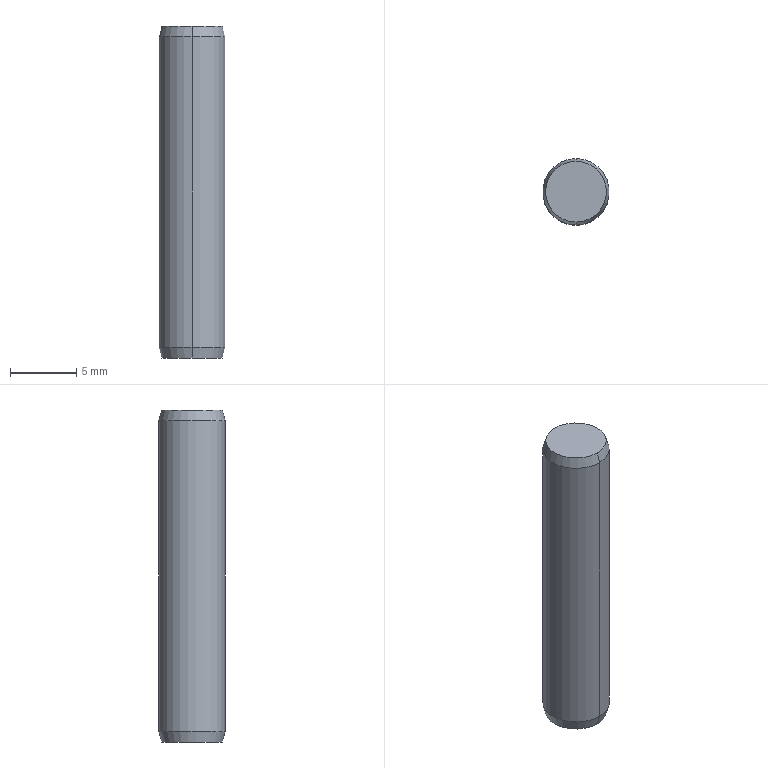Component | NX | PIN_M5X25 | 1 solid | 8 faces | box 5 x 5 x 25 mm | volume 488 mm3 | cone 4 | cylinder 2 | plane 2 | commonest cylinder face diameters 5 x2
STEP:
#1=CARTESIAN_POINT('',(0.,0.,0.));
#2=DIRECTION('',(0.,0.,1.));
#3=DIRECTION('',(1.,0.,0.));
#4=AXIS2_PLACEMENT_3D('',#1,#2,#3);
#5=CARTESIAN_POINT('',(-222.594,88.985,75.8));
#6=VERTEX_POINT('',#5);
#7=CARTESIAN_POINT('',(-222.594,88.77,75.));
#8=VERTEX_POINT('',#7);
#9=CARTESIAN_POINT('',(-222.594,88.878,75.4));
#10=DIRECTION('',(0.,-0.2588,-0.9659));
#11=VECTOR('',#10,1.);
#12=LINE('',#9,#11);
#13=CARTESIAN_POINT('',(-222.594,86.485,75.4));
#14=DIRECTION('',(0.,0.,1.));
#15=DIRECTION('',(0.,-1.,0.));
#16=AXIS2_PLACEMENT_3D('',#13,#14,#15);
#17=CONICAL_SURFACE('',#16,2.393,0.2618);
#18=CARTESIAN_POINT('',(3.142,-0.));
#19=DIRECTION('',(0.,-1.));
#20=VECTOR('',#19,1.);
#21=LINE('',#18,#20);
#22=(GEOMETRIC_REPRESENTATION_CONTEXT(2)PARAMETRIC_REPRESENTATION_CONTEXT()REPRESENTATION_CONTEXT('',''));
#23=DEFINITIONAL_REPRESENTATION('',(#21),#22);
#24=PCURVE('',#17,#23);
#25=CARTESIAN_POINT('',(-222.594,86.485,75.4));
#26=DIRECTION('',(0.,0.,1.));
#27=DIRECTION('',(0.,-1.,0.));
#28=AXIS2_PLACEMENT_3D('',#25,#26,#27);
#29=CONICAL_SURFACE('',#28,2.393,0.2618);
#30=CARTESIAN_POINT('',(3.142,-0.));
#31=DIRECTION('',(0.,-1.));
#32=VECTOR('',#31,1.);
#33=LINE('',#30,#32);
#34=(GEOMETRIC_REPRESENTATION_CONTEXT(2)PARAMETRIC_REPRESENTATION_CONTEXT()REPRESENTATION_CONTEXT('',''));
#35=DEFINITIONAL_REPRESENTATION('',(#33),#34);
#36=PCURVE('',#29,#35);
#37=SURFACE_CURVE('',#12,(#24,#36),.PCURVE_S1.);
#38=EDGE_CURVE('',#6,#8,#37,.T.);
#39=ORIENTED_EDGE('',*,*,#38,.F.);
#40=CARTESIAN_POINT('',(-222.594,83.985,75.8));
#41=VERTEX_POINT('',#40);
#42=CARTESIAN_POINT('',(-222.594,86.485,75.8));
#43=DIRECTION('',(0.,0.,-1.));
#44=DIRECTION('',(0.,1.,0.));
#45=AXIS2_PLACEMENT_3D('',#42,#43,#44);
#46=CIRCLE('',#45,2.5);
#47=CARTESIAN_POINT('',(3.142,0.4));
#48=DIRECTION('',(-1.,0.));
#49=VECTOR('',#48,1.);
#50=LINE('',#47,#49);
#51=(GEOMETRIC_REPRESENTATION_CONTEXT(2)PARAMETRIC_REPRESENTATION_CONTEXT()REPRESENTATION_CONTEXT('',''));
#52=DEFINITIONAL_REPRESENTATION('',(#50),#51);
#53=PCURVE('',#17,#52);
#54=CARTESIAN_POINT('',(-222.594,86.485,90.));
#55=DIRECTION('',(0.,0.,-1.));
#56=DIRECTION('',(0.,-1.,0.));
#57=AXIS2_PLACEMENT_3D('',#54,#55,#56);
#58=CYLINDRICAL_SURFACE('',#57,2.5);
#59=CARTESIAN_POINT('',(3.142,14.2));
#60=DIRECTION('',(1.,0.));
#61=VECTOR('',#60,1.);
#62=LINE('',#59,#61);
#63=(GEOMETRIC_REPRESENTATION_CONTEXT(2)PARAMETRIC_REPRESENTATION_CONTEXT()REPRESENTATION_CONTEXT('',''));
#64=DEFINITIONAL_REPRESENTATION('',(#62),#63);
#65=PCURVE('',#58,#64);
#66=SURFACE_CURVE('',#46,(#53,#65),.PCURVE_S1.);
#67=EDGE_CURVE('',#6,#41,#66,.T.);
#68=ORIENTED_EDGE('',*,*,#67,.T.);
#69=CARTESIAN_POINT('',(-222.594,84.199,75.));
#70=VERTEX_POINT('',#69);
#71=CARTESIAN_POINT('',(-222.594,84.092,75.4));
#72=DIRECTION('',(0.,-0.2588,0.9659));
#73=VECTOR('',#72,1.);
#74=LINE('',#71,#73);
#75=CARTESIAN_POINT('',(0.,0.));
#76=DIRECTION('',(0.,1.));
#77=VECTOR('',#76,1.);
#78=LINE('',#75,#77);
#79=(GEOMETRIC_REPRESENTATION_CONTEXT(2)PARAMETRIC_REPRESENTATION_CONTEXT()REPRESENTATION_CONTEXT('',''));
#80=DEFINITIONAL_REPRESENTATION('',(#78),#79);
#81=PCURVE('',#17,#80);
#82=CARTESIAN_POINT('',(6.283,0.));
#83=DIRECTION('',(0.,1.));
#84=VECTOR('',#83,1.);
#85=LINE('',#82,#84);
#86=(GEOMETRIC_REPRESENTATION_CONTEXT(2)PARAMETRIC_REPRESENTATION_CONTEXT()REPRESENTATION_CONTEXT('',''));
#87=DEFINITIONAL_REPRESENTATION('',(#85),#86);
#88=PCURVE('',#29,#87);
#89=SURFACE_CURVE('',#74,(#81,#88),.PCURVE_S1.);
#90=EDGE_CURVE('',#70,#41,#89,.T.);
#91=ORIENTED_EDGE('',*,*,#90,.F.);
#92=CARTESIAN_POINT('',(-222.594,86.485,75.));
#93=DIRECTION('',(0.,0.,-1.));
#94=DIRECTION('',(0.,1.,0.));
#95=AXIS2_PLACEMENT_3D('',#92,#93,#94);
#96=CIRCLE('',#95,2.286);
#97=CARTESIAN_POINT('',(3.142,-0.4));
#98=DIRECTION('',(-1.,0.));
#99=VECTOR('',#98,1.);
#100=LINE('',#97,#99);
#101=(GEOMETRIC_REPRESENTATION_CONTEXT(2)PARAMETRIC_REPRESENTATION_CONTEXT()REPRESENTATION_CONTEXT('',''));
#102=DEFINITIONAL_REPRESENTATION('',(#100),#101);
#103=PCURVE('',#17,#102);
#104=CARTESIAN_POINT('',(-222.594,87.628,75.));
#105=DIRECTION('',(0.,0.,-1.));
#106=DIRECTION('',(0.,-1.,0.));
#107=AXIS2_PLACEMENT_3D('',#104,#105,#106);
#108=PLANE('',#107);
#109=CARTESIAN_POINT('',(1.143,0.));
#110=DIRECTION('',(-1.,0.));
#111=AXIS2_PLACEMENT_2D('',#109,#110);
#112=CIRCLE('',#111,2.286);
#113=(GEOMETRIC_REPRESENTATION_CONTEXT(2)PARAMETRIC_REPRESENTATION_CONTEXT()REPRESENTATION_CONTEXT('',''));
#114=DEFINITIONAL_REPRESENTATION('',(#112),#113);
#115=PCURVE('',#108,#114);
#116=SURFACE_CURVE('',#96,(#103,#115),.PCURVE_S1.);
#117=EDGE_CURVE('',#8,#70,#116,.T.);
#118=ORIENTED_EDGE('',*,*,#117,.F.);
#119=EDGE_LOOP('',(#39,#68,#91,#118));
#120=FACE_BOUND('',#119,.T.);
#121=ADVANCED_FACE('',(#120),#17,.T.);
#122=CARTESIAN_POINT('',(-222.594,88.985,99.2));
#123=VERTEX_POINT('',#122);
#124=CARTESIAN_POINT('',(-222.594,88.985,90.));
#125=DIRECTION('',(0.,0.,-1.));
#126=VECTOR('',#125,1.);
#127=LINE('',#124,#126);
#128=CARTESIAN_POINT('',(3.142,0.));
#129=DIRECTION('',(0.,1.));
#130=VECTOR('',#129,1.);
#131=LINE('',#128,#130);
#132=(GEOMETRIC_REPRESENTATION_CONTEXT(2)PARAMETRIC_REPRESENTATION_CONTEXT()REPRESENTATION_CONTEXT('',''));
#133=DEFINITIONAL_REPRESENTATION('',(#131),#132);
#134=PCURVE('',#58,#133);
#135=CARTESIAN_POINT('',(-222.594,86.485,90.));
#136=DIRECTION('',(0.,0.,-1.));
#137=DIRECTION('',(0.,-1.,0.));
#138=AXIS2_PLACEMENT_3D('',#135,#136,#137);
#139=CYLINDRICAL_SURFACE('',#138,2.5);
#140=CARTESIAN_POINT('',(3.142,0.));
#141=DIRECTION('',(0.,1.));
#142=VECTOR('',#141,1.);
#143=LINE('',#140,#142);
#144=(GEOMETRIC_REPRESENTATION_CONTEXT(2)PARAMETRIC_REPRESENTATION_CONTEXT()REPRESENTATION_CONTEXT('',''));
#145=DEFINITIONAL_REPRESENTATION('',(#143),#144);
#146=PCURVE('',#139,#145);
#147=SURFACE_CURVE('',#127,(#134,#146),.PCURVE_S1.);
#148=EDGE_CURVE('',#123,#6,#147,.T.);
#149=ORIENTED_EDGE('',*,*,#148,.F.);
#150=CARTESIAN_POINT('',(-222.594,83.985,99.2));
#151=VERTEX_POINT('',#150);
#152=CARTESIAN_POINT('',(-222.594,86.485,99.2));
#153=DIRECTION('',(0.,0.,-1.));
#154=DIRECTION('',(0.,1.,0.));
#155=AXIS2_PLACEMENT_3D('',#152,#153,#154);
#156=CIRCLE('',#155,2.5);
#157=CARTESIAN_POINT('',(3.142,-9.2));
#158=DIRECTION('',(1.,0.));
#159=VECTOR('',#158,1.);
#160=LINE('',#157,#159);
#161=(GEOMETRIC_REPRESENTATION_CONTEXT(2)PARAMETRIC_REPRESENTATION_CONTEXT()REPRESENTATION_CONTEXT('',''));
#162=DEFINITIONAL_REPRESENTATION('',(#160),#161);
#163=PCURVE('',#58,#162);
#164=CARTESIAN_POINT('',(-222.594,86.485,99.6));
#165=DIRECTION('',(0.,0.,-1.));
#166=DIRECTION('',(0.,-1.,0.));
#167=AXIS2_PLACEMENT_3D('',#164,#165,#166);
#168=CONICAL_SURFACE('',#167,2.393,0.2618);
#169=CARTESIAN_POINT('',(3.142,0.4));
#170=DIRECTION('',(1.,0.));
#171=VECTOR('',#170,1.);
#172=LINE('',#169,#171);
#173=(GEOMETRIC_REPRESENTATION_CONTEXT(2)PARAMETRIC_REPRESENTATION_CONTEXT()REPRESENTATION_CONTEXT('',''));
#174=DEFINITIONAL_REPRESENTATION('',(#172),#173);
#175=PCURVE('',#168,#174);
#176=SURFACE_CURVE('',#156,(#163,#175),.PCURVE_S1.);
#177=EDGE_CURVE('',#123,#151,#176,.T.);
#178=ORIENTED_EDGE('',*,*,#177,.T.);
#179=CARTESIAN_POINT('',(-222.594,83.985,90.));
#180=DIRECTION('',(0.,0.,1.));
#181=VECTOR('',#180,1.);
#182=LINE('',#179,#181);
#183=CARTESIAN_POINT('',(6.283,0.));
#184=DIRECTION('',(0.,-1.));
#185=VECTOR('',#184,1.);
#186=LINE('',#183,#185);
#187=(GEOMETRIC_REPRESENTATION_CONTEXT(2)PARAMETRIC_REPRESENTATION_CONTEXT()REPRESENTATION_CONTEXT('',''));
#188=DEFINITIONAL_REPRESENTATION('',(#186),#187);
#189=PCURVE('',#58,#188);
#190=CARTESIAN_POINT('',(0.,0.));
#191=DIRECTION('',(0.,-1.));
#192=VECTOR('',#191,1.);
#193=LINE('',#190,#192);
#194=(GEOMETRIC_REPRESENTATION_CONTEXT(2)PARAMETRIC_REPRESENTATION_CONTEXT()REPRESENTATION_CONTEXT('',''));
#195=DEFINITIONAL_REPRESENTATION('',(#193),#194);
#196=PCURVE('',#139,#195);
#197=SURFACE_CURVE('',#182,(#189,#196),.PCURVE_S1.);
#198=EDGE_CURVE('',#41,#151,#197,.T.);
#199=ORIENTED_EDGE('',*,*,#198,.F.);
#200=ORIENTED_EDGE('',*,*,#67,.F.);
#201=EDGE_LOOP('',(#149,#178,#199,#200));
#202=FACE_BOUND('',#201,.T.);
#203=ADVANCED_FACE('',(#202),#58,.T.);
#204=CARTESIAN_POINT('',(-222.594,88.77,100.));
#205=VERTEX_POINT('',#204);
#206=CARTESIAN_POINT('',(-222.594,88.878,99.6));
#207=DIRECTION('',(-0.,0.2588,-0.9659));
#208=VECTOR('',#207,1.);
#209=LINE('',#206,#208);
#210=CARTESIAN_POINT('',(3.142,-0.));
#211=DIRECTION('',(0.,1.));
#212=VECTOR('',#211,1.);
#213=LINE('',#210,#212);
#214=(GEOMETRIC_REPRESENTATION_CONTEXT(2)PARAMETRIC_REPRESENTATION_CONTEXT()REPRESENTATION_CONTEXT('',''));
#215=DEFINITIONAL_REPRESENTATION('',(#213),#214);
#216=PCURVE('',#168,#215);
#217=CARTESIAN_POINT('',(-222.594,86.485,99.6));
#218=DIRECTION('',(0.,0.,-1.));
#219=DIRECTION('',(0.,-1.,0.));
#220=AXIS2_PLACEMENT_3D('',#217,#218,#219);
#221=CONICAL_SURFACE('',#220,2.393,0.2618);
#222=CARTESIAN_POINT('',(3.142,-0.));
#223=DIRECTION('',(0.,1.));
#224=VECTOR('',#223,1.);
#225=LINE('',#222,#224);
#226=(GEOMETRIC_REPRESENTATION_CONTEXT(2)PARAMETRIC_REPRESENTATION_CONTEXT()REPRESENTATION_CONTEXT('',''));
#227=DEFINITIONAL_REPRESENTATION('',(#225),#226);
#228=PCURVE('',#221,#227);
#229=SURFACE_CURVE('',#209,(#216,#228),.PCURVE_S1.);
#230=EDGE_CURVE('',#205,#123,#229,.T.);
#231=ORIENTED_EDGE('',*,*,#230,.F.);
#232=CARTESIAN_POINT('',(-222.594,84.199,100.));
#233=VERTEX_POINT('',#232);
#234=CARTESIAN_POINT('',(-222.594,86.485,100.));
#235=DIRECTION('',(0.,0.,-1.));
#236=DIRECTION('',(0.,1.,0.));
#237=AXIS2_PLACEMENT_3D('',#234,#235,#236);
#238=CIRCLE('',#237,2.286);
#239=CARTESIAN_POINT('',(3.142,-0.4));
#240=DIRECTION('',(1.,0.));
#241=VECTOR('',#240,1.);
#242=LINE('',#239,#241);
#243=(GEOMETRIC_REPRESENTATION_CONTEXT(2)PARAMETRIC_REPRESENTATION_CONTEXT()REPRESENTATION_CONTEXT('',''));
#244=DEFINITIONAL_REPRESENTATION('',(#242),#243);
#245=PCURVE('',#168,#244);
#246=CARTESIAN_POINT('',(-222.594,87.628,100.));
#247=DIRECTION('',(0.,0.,1.));
#248=DIRECTION('',(0.,1.,0.));
#249=AXIS2_PLACEMENT_3D('',#246,#247,#248);
#250=PLANE('',#249);
#251=CARTESIAN_POINT('',(1.143,0.));
#252=CARTESIAN_POINT('',(1.143,-3.959));
#253=CARTESIAN_POINT('',(-2.286,-1.979));
#254=CARTESIAN_POINT('',(-5.714,-0.));
#255=CARTESIAN_POINT('',(-2.286,1.979));
#256=CARTESIAN_POINT('',(1.143,3.959));
#257=CARTESIAN_POINT('',(1.143,0.));
#258=(BOUNDED_CURVE()B_SPLINE_CURVE(2,(#251,#252,#253,#254,#255,#256,#257),.UNSPECIFIED.,.T.,.F.)B_SPLINE_CURVE_WITH_KNOTS((1,2,2,2,2,1),(-2.094,0.,2.094,4.189,6.283,8.378),.UNSPECIFIED.)CURVE()GEOMETRIC_REPRESENTATION_ITEM()RATIONAL_B_SPLINE_CURVE((1.,0.5,1.,0.5,1.,0.5,1.))REPRESENTATION_ITEM(''));
#259=(GEOMETRIC_REPRESENTATION_CONTEXT(2)PARAMETRIC_REPRESENTATION_CONTEXT()REPRESENTATION_CONTEXT('',''));
#260=DEFINITIONAL_REPRESENTATION('',(#258),#259);
#261=PCURVE('',#250,#260);
#262=SURFACE_CURVE('',#238,(#245,#261),.PCURVE_S1.);
#263=EDGE_CURVE('',#205,#233,#262,.T.);
#264=ORIENTED_EDGE('',*,*,#263,.T.);
#265=CARTESIAN_POINT('',(-222.594,84.092,99.6));
#266=DIRECTION('',(-0.,0.2588,0.9659));
#267=VECTOR('',#266,1.);
#268=LINE('',#265,#267);
#269=CARTESIAN_POINT('',(6.283,0.));
#270=DIRECTION('',(0.,-1.));
#271=VECTOR('',#270,1.);
#272=LINE('',#269,#271);
#273=(GEOMETRIC_REPRESENTATION_CONTEXT(2)PARAMETRIC_REPRESENTATION_CONTEXT()REPRESENTATION_CONTEXT('',''));
#274=DEFINITIONAL_REPRESENTATION('',(#272),#273);
#275=PCURVE('',#168,#274);
#276=CARTESIAN_POINT('',(0.,0.));
#277=DIRECTION('',(0.,-1.));
#278=VECTOR('',#277,1.);
#279=LINE('',#276,#278);
#280=(GEOMETRIC_REPRESENTATION_CONTEXT(2)PARAMETRIC_REPRESENTATION_CONTEXT()REPRESENTATION_CONTEXT('',''));
#281=DEFINITIONAL_REPRESENTATION('',(#279),#280);
#282=PCURVE('',#221,#281);
#283=SURFACE_CURVE('',#268,(#275,#282),.PCURVE_S1.);
#284=EDGE_CURVE('',#151,#233,#283,.T.);
#285=ORIENTED_EDGE('',*,*,#284,.F.);
#286=ORIENTED_EDGE('',*,*,#177,.F.);
#287=EDGE_LOOP('',(#231,#264,#285,#286));
#288=FACE_BOUND('',#287,.T.);
#289=ADVANCED_FACE('',(#288),#168,.T.);
#290=ORIENTED_EDGE('',*,*,#230,.T.);
#291=CARTESIAN_POINT('',(-222.594,86.485,99.2));
#292=DIRECTION('',(0.,0.,-1.));
#293=DIRECTION('',(0.,1.,0.));
#294=AXIS2_PLACEMENT_3D('',#291,#292,#293);
#295=CIRCLE('',#294,2.5);
#296=CARTESIAN_POINT('',(-3.142,0.4));
#297=DIRECTION('',(1.,0.));
#298=VECTOR('',#297,1.);
#299=LINE('',#296,#298);
#300=(GEOMETRIC_REPRESENTATION_CONTEXT(2)PARAMETRIC_REPRESENTATION_CONTEXT()REPRESENTATION_CONTEXT('',''));
#301=DEFINITIONAL_REPRESENTATION('',(#299),#300);
#302=PCURVE('',#221,#301);
#303=CARTESIAN_POINT('',(-3.142,-9.2));
#304=DIRECTION('',(1.,0.));
#305=VECTOR('',#304,1.);
#306=LINE('',#303,#305);
#307=(GEOMETRIC_REPRESENTATION_CONTEXT(2)PARAMETRIC_REPRESENTATION_CONTEXT()REPRESENTATION_CONTEXT('',''));
#308=DEFINITIONAL_REPRESENTATION('',(#306),#307);
#309=PCURVE('',#139,#308);
#310=SURFACE_CURVE('',#295,(#302,#309),.PCURVE_S1.);
#311=EDGE_CURVE('',#151,#123,#310,.T.);
#312=ORIENTED_EDGE('',*,*,#311,.F.);
#313=ORIENTED_EDGE('',*,*,#284,.T.);
#314=CARTESIAN_POINT('',(-222.594,86.485,100.));
#315=DIRECTION('',(0.,0.,-1.));
#316=DIRECTION('',(0.,1.,0.));
#317=AXIS2_PLACEMENT_3D('',#314,#315,#316);
#318=CIRCLE('',#317,2.286);
#319=CARTESIAN_POINT('',(-3.142,-0.4));
#320=DIRECTION('',(1.,0.));
#321=VECTOR('',#320,1.);
#322=LINE('',#319,#321);
#323=(GEOMETRIC_REPRESENTATION_CONTEXT(2)PARAMETRIC_REPRESENTATION_CONTEXT()REPRESENTATION_CONTEXT('',''));
#324=DEFINITIONAL_REPRESENTATION('',(#322),#323);
#325=PCURVE('',#221,#324);
#326=CARTESIAN_POINT('',(1.143,0.));
#327=CARTESIAN_POINT('',(1.143,-3.959));
#328=CARTESIAN_POINT('',(-2.286,-1.979));
#329=CARTESIAN_POINT('',(-5.714,-0.));
#330=CARTESIAN_POINT('',(-2.286,1.979));
#331=CARTESIAN_POINT('',(1.143,3.959));
#332=CARTESIAN_POINT('',(1.143,0.));
#333=(BOUNDED_CURVE()B_SPLINE_CURVE(2,(#326,#327,#328,#329,#330,#331,#332),.UNSPECIFIED.,.T.,.F.)B_SPLINE_CURVE_WITH_KNOTS((1,2,2,2,2,1),(-2.094,0.,2.094,4.189,6.283,8.378),.UNSPECIFIED.)CURVE()GEOMETRIC_REPRESENTATION_ITEM()RATIONAL_B_SPLINE_CURVE((1.,0.5,1.,0.5,1.,0.5,1.))REPRESENTATION_ITEM(''));
#334=(GEOMETRIC_REPRESENTATION_CONTEXT(2)PARAMETRIC_REPRESENTATION_CONTEXT()REPRESENTATION_CONTEXT('',''));
#335=DEFINITIONAL_REPRESENTATION('',(#333),#334);
#336=PCURVE('',#250,#335);
#337=SURFACE_CURVE('',#318,(#325,#336),.PCURVE_S1.);
#338=EDGE_CURVE('',#233,#205,#337,.T.);
#339=ORIENTED_EDGE('',*,*,#338,.T.);
#340=EDGE_LOOP('',(#290,#312,#313,#339));
#341=FACE_BOUND('',#340,.T.);
#342=ADVANCED_FACE('',(#341),#221,.T.);
#343=ORIENTED_EDGE('',*,*,#148,.T.);
#344=CARTESIAN_POINT('',(-222.594,86.485,75.8));
#345=DIRECTION('',(0.,0.,-1.));
#346=DIRECTION('',(0.,1.,0.));
#347=AXIS2_PLACEMENT_3D('',#344,#345,#346);
#348=CIRCLE('',#347,2.5);
#349=CARTESIAN_POINT('',(-3.142,14.2));
#350=DIRECTION('',(1.,0.));
#351=VECTOR('',#350,1.);
#352=LINE('',#349,#351);
#353=(GEOMETRIC_REPRESENTATION_CONTEXT(2)PARAMETRIC_REPRESENTATION_CONTEXT()REPRESENTATION_CONTEXT('',''));
#354=DEFINITIONAL_REPRESENTATION('',(#352),#353);
#355=PCURVE('',#139,#354);
#356=CARTESIAN_POINT('',(9.425,0.4));
#357=DIRECTION('',(-1.,0.));
#358=VECTOR('',#357,1.);
#359=LINE('',#356,#358);
#360=(GEOMETRIC_REPRESENTATION_CONTEXT(2)PARAMETRIC_REPRESENTATION_CONTEXT()REPRESENTATION_CONTEXT('',''));
#361=DEFINITIONAL_REPRESENTATION('',(#359),#360);
#362=PCURVE('',#29,#361);
#363=SURFACE_CURVE('',#348,(#355,#362),.PCURVE_S1.);
#364=EDGE_CURVE('',#41,#6,#363,.T.);
#365=ORIENTED_EDGE('',*,*,#364,.F.);
#366=ORIENTED_EDGE('',*,*,#198,.T.);
#367=ORIENTED_EDGE('',*,*,#311,.T.);
#368=EDGE_LOOP('',(#343,#365,#366,#367));
#369=FACE_BOUND('',#368,.T.);
#370=ADVANCED_FACE('',(#369),#139,.T.);
#371=ORIENTED_EDGE('',*,*,#38,.T.);
#372=CARTESIAN_POINT('',(-222.594,86.485,75.));
#373=DIRECTION('',(0.,0.,-1.));
#374=DIRECTION('',(0.,1.,0.));
#375=AXIS2_PLACEMENT_3D('',#372,#373,#374);
#376=CIRCLE('',#375,2.286);
#377=CARTESIAN_POINT('',(9.425,-0.4));
#378=DIRECTION('',(-1.,0.));
#379=VECTOR('',#378,1.);
#380=LINE('',#377,#379);
#381=(GEOMETRIC_REPRESENTATION_CONTEXT(2)PARAMETRIC_REPRESENTATION_CONTEXT()REPRESENTATION_CONTEXT('',''));
#382=DEFINITIONAL_REPRESENTATION('',(#380),#381);
#383=PCURVE('',#29,#382);
#384=CARTESIAN_POINT('',(1.143,0.));
#385=DIRECTION('',(-1.,0.));
#386=AXIS2_PLACEMENT_2D('',#384,#385);
#387=CIRCLE('',#386,2.286);
#388=(GEOMETRIC_REPRESENTATION_CONTEXT(2)PARAMETRIC_REPRESENTATION_CONTEXT()REPRESENTATION_CONTEXT('',''));
#389=DEFINITIONAL_REPRESENTATION('',(#387),#388);
#390=PCURVE('',#108,#389);
#391=SURFACE_CURVE('',#376,(#383,#390),.PCURVE_S1.);
#392=EDGE_CURVE('',#70,#8,#391,.T.);
#393=ORIENTED_EDGE('',*,*,#392,.F.);
#394=ORIENTED_EDGE('',*,*,#90,.T.);
#395=ORIENTED_EDGE('',*,*,#364,.T.);
#396=EDGE_LOOP('',(#371,#393,#394,#395));
#397=FACE_BOUND('',#396,.T.);
#398=ADVANCED_FACE('',(#397),#29,.T.);
#399=ORIENTED_EDGE('',*,*,#117,.T.);
#400=ORIENTED_EDGE('',*,*,#392,.T.);
#401=EDGE_LOOP('',(#399,#400));
#402=FACE_BOUND('',#401,.T.);
#403=ADVANCED_FACE('',(#402),#108,.T.);
#404=ORIENTED_EDGE('',*,*,#263,.F.);
#405=ORIENTED_EDGE('',*,*,#338,.F.);
#406=EDGE_LOOP('',(#404,#405));
#407=FACE_BOUND('',#406,.T.);
#408=ADVANCED_FACE('',(#407),#250,.T.);
#409=CLOSED_SHELL('',(#121,#203,#289,#342,#370,#398,#403,#408));
#410=MANIFOLD_SOLID_BREP('',#409);
#411=(LENGTH_UNIT()NAMED_UNIT(*)SI_UNIT(.MILLI.,.METRE.));
#412=UNCERTAINTY_MEASURE_WITH_UNIT(LENGTH_MEASURE(0.0000001),#411,'','');
#413=(NAMED_UNIT(*)PLANE_ANGLE_UNIT()SI_UNIT($,.RADIAN.));
#414=(NAMED_UNIT(*)SI_UNIT($,.STERADIAN.)SOLID_ANGLE_UNIT());
#415=(GEOMETRIC_REPRESENTATION_CONTEXT(3)GLOBAL_UNCERTAINTY_ASSIGNED_CONTEXT((#412))GLOBAL_UNIT_ASSIGNED_CONTEXT((#411,#413,#414))REPRESENTATION_CONTEXT('',''));
#416=ADVANCED_BREP_SHAPE_REPRESENTATION('',(#4,#410),#415);